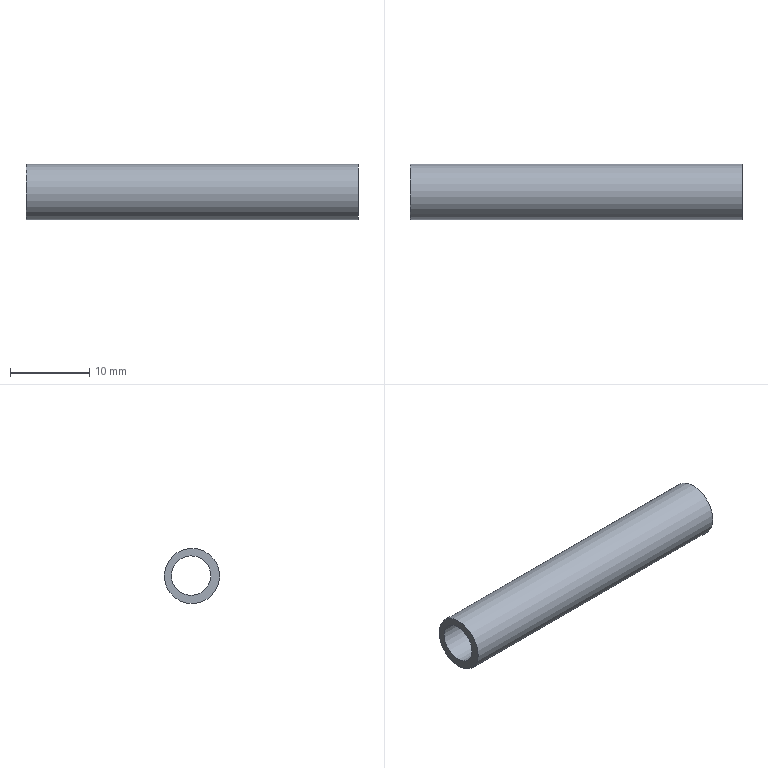Component | NX | 23F__27 | 1 solid | 4 faces | box 42 x 7 x 7 mm | volume 792 mm3 | cylinder 2 | plane 2 | commonest cylinder face diameters 7 x1 5 x1
STEP:
#1=CARTESIAN_POINT('',(0.,0.,0.));
#2=DIRECTION('',(0.,0.,1.));
#3=DIRECTION('',(1.,0.,0.));
#4=AXIS2_PLACEMENT_3D('',#1,#2,#3);
#5=CARTESIAN_POINT('',(87.522,47.062,142.252));
#6=VERTEX_POINT('',#5);
#7=CARTESIAN_POINT('',(87.522,45.581,145.424));
#8=DIRECTION('',(1.,0.,0.));
#9=DIRECTION('',(0.,0.4231,-0.9061));
#10=AXIS2_PLACEMENT_3D('',#7,#8,#9);
#11=CIRCLE('',#10,3.5);
#12=CARTESIAN_POINT('',(87.522,45.581,145.424));
#13=DIRECTION('',(-1.,0.,0.));
#14=DIRECTION('',(0.,-0.4231,0.9061));
#15=AXIS2_PLACEMENT_3D('',#12,#13,#14);
#16=CYLINDRICAL_SURFACE('',#15,3.5);
#17=CARTESIAN_POINT('',(9.425,0.));
#18=DIRECTION('',(-1.,0.));
#19=VECTOR('',#18,1.);
#20=LINE('',#17,#19);
#21=(GEOMETRIC_REPRESENTATION_CONTEXT(2)PARAMETRIC_REPRESENTATION_CONTEXT()REPRESENTATION_CONTEXT('',''));
#22=DEFINITIONAL_REPRESENTATION('',(#20),#21);
#23=PCURVE('',#16,#22);
#24=CARTESIAN_POINT('',(87.522,45.639,145.451));
#25=DIRECTION('',(1.,0.,0.));
#26=DIRECTION('',(0.,0.4231,-0.9061));
#27=AXIS2_PLACEMENT_3D('',#24,#25,#26);
#28=PLANE('',#27);
#29=CARTESIAN_POINT('',(0.,-0.06341));
#30=DIRECTION('',(1.,0.));
#31=AXIS2_PLACEMENT_2D('',#29,#30);
#32=CIRCLE('',#31,3.5);
#33=(GEOMETRIC_REPRESENTATION_CONTEXT(2)PARAMETRIC_REPRESENTATION_CONTEXT()REPRESENTATION_CONTEXT('',''));
#34=DEFINITIONAL_REPRESENTATION('',(#32),#33);
#35=PCURVE('',#28,#34);
#36=SURFACE_CURVE('',#11,(#23,#35),.PCURVE_S1.);
#37=EDGE_CURVE('',#6,#6,#36,.T.);
#38=ORIENTED_EDGE('',*,*,#37,.F.);
#39=CARTESIAN_POINT('',(45.522,47.062,142.252));
#40=VERTEX_POINT('',#39);
#41=CARTESIAN_POINT('',(87.522,47.062,142.252));
#42=CARTESIAN_POINT('',(45.522,47.062,142.252));
#43=B_SPLINE_CURVE_WITH_KNOTS('',1,(#41,#42),.UNSPECIFIED.,.F.,.F.,(2,2),(0.,42.),.PIECEWISE_BEZIER_KNOTS.);
#44=CARTESIAN_POINT('',(9.425,0.));
#45=DIRECTION('',(0.,1.));
#46=VECTOR('',#45,1.);
#47=LINE('',#44,#46);
#48=(GEOMETRIC_REPRESENTATION_CONTEXT(2)PARAMETRIC_REPRESENTATION_CONTEXT()REPRESENTATION_CONTEXT('',''));
#49=DEFINITIONAL_REPRESENTATION('',(#47),#48);
#50=PCURVE('',#16,#49);
#51=CARTESIAN_POINT('',(3.142,0.));
#52=DIRECTION('',(0.,1.));
#53=VECTOR('',#52,1.);
#54=LINE('',#51,#53);
#55=(GEOMETRIC_REPRESENTATION_CONTEXT(2)PARAMETRIC_REPRESENTATION_CONTEXT()REPRESENTATION_CONTEXT('',''));
#56=DEFINITIONAL_REPRESENTATION('',(#54),#55);
#57=PCURVE('',#16,#56);
#58=SEAM_CURVE('',#43,(#50,#57),.PCURVE_S1.);
#59=EDGE_CURVE('',#6,#40,#58,.T.);
#60=ORIENTED_EDGE('',*,*,#59,.T.);
#61=CARTESIAN_POINT('',(45.522,45.581,145.424));
#62=DIRECTION('',(1.,0.,0.));
#63=DIRECTION('',(0.,0.4231,-0.9061));
#64=AXIS2_PLACEMENT_3D('',#61,#62,#63);
#65=CIRCLE('',#64,3.5);
#66=CARTESIAN_POINT('',(9.425,42.));
#67=DIRECTION('',(-1.,0.));
#68=VECTOR('',#67,1.);
#69=LINE('',#66,#68);
#70=(GEOMETRIC_REPRESENTATION_CONTEXT(2)PARAMETRIC_REPRESENTATION_CONTEXT()REPRESENTATION_CONTEXT('',''));
#71=DEFINITIONAL_REPRESENTATION('',(#69),#70);
#72=PCURVE('',#16,#71);
#73=CARTESIAN_POINT('',(45.522,45.639,145.451));
#74=DIRECTION('',(1.,0.,0.));
#75=DIRECTION('',(0.,0.4231,-0.9061));
#76=AXIS2_PLACEMENT_3D('',#73,#74,#75);
#77=PLANE('',#76);
#78=CARTESIAN_POINT('',(0.,-0.06341));
#79=DIRECTION('',(1.,0.));
#80=AXIS2_PLACEMENT_2D('',#78,#79);
#81=CIRCLE('',#80,3.5);
#82=(GEOMETRIC_REPRESENTATION_CONTEXT(2)PARAMETRIC_REPRESENTATION_CONTEXT()REPRESENTATION_CONTEXT('',''));
#83=DEFINITIONAL_REPRESENTATION('',(#81),#82);
#84=PCURVE('',#77,#83);
#85=SURFACE_CURVE('',#65,(#72,#84),.PCURVE_S1.);
#86=EDGE_CURVE('',#40,#40,#85,.T.);
#87=ORIENTED_EDGE('',*,*,#86,.T.);
#88=ORIENTED_EDGE('',*,*,#59,.F.);
#89=EDGE_LOOP('',(#38,#60,#87,#88));
#90=FACE_BOUND('',#89,.T.);
#91=ADVANCED_FACE('',(#90),#16,.T.);
#92=CARTESIAN_POINT('',(87.522,46.754,143.212));
#93=VERTEX_POINT('',#92);
#94=CARTESIAN_POINT('',(87.522,45.696,145.477));
#95=DIRECTION('',(-1.,0.,0.));
#96=DIRECTION('',(0.,0.4231,-0.9061));
#97=AXIS2_PLACEMENT_3D('',#94,#95,#96);
#98=CIRCLE('',#97,2.5);
#99=CARTESIAN_POINT('',(87.522,45.696,145.477));
#100=DIRECTION('',(-1.,0.,0.));
#101=DIRECTION('',(0.,-0.4231,0.9061));
#102=AXIS2_PLACEMENT_3D('',#99,#100,#101);
#103=CYLINDRICAL_SURFACE('',#102,2.5);
#104=CARTESIAN_POINT('',(3.142,0.));
#105=DIRECTION('',(1.,0.));
#106=VECTOR('',#105,1.);
#107=LINE('',#104,#106);
#108=(GEOMETRIC_REPRESENTATION_CONTEXT(2)PARAMETRIC_REPRESENTATION_CONTEXT()REPRESENTATION_CONTEXT('',''));
#109=DEFINITIONAL_REPRESENTATION('',(#107),#108);
#110=PCURVE('',#103,#109);
#111=CARTESIAN_POINT('',(2.5,0.06341));
#112=CARTESIAN_POINT('',(2.5,-4.267));
#113=CARTESIAN_POINT('',(-1.25,-2.102));
#114=CARTESIAN_POINT('',(-5.,0.06341));
#115=CARTESIAN_POINT('',(-1.25,2.228));
#116=CARTESIAN_POINT('',(2.5,4.394));
#117=CARTESIAN_POINT('',(2.5,0.06341));
#118=(BOUNDED_CURVE()B_SPLINE_CURVE(2,(#111,#112,#113,#114,#115,#116,#117),.UNSPECIFIED.,.T.,.F.)B_SPLINE_CURVE_WITH_KNOTS((1,2,2,2,2,1),(-2.094,0.,2.094,4.189,6.283,8.378),.UNSPECIFIED.)CURVE()GEOMETRIC_REPRESENTATION_ITEM()RATIONAL_B_SPLINE_CURVE((1.,0.5,1.,0.5,1.,0.5,1.))REPRESENTATION_ITEM(''));
#119=(GEOMETRIC_REPRESENTATION_CONTEXT(2)PARAMETRIC_REPRESENTATION_CONTEXT()REPRESENTATION_CONTEXT('',''));
#120=DEFINITIONAL_REPRESENTATION('',(#118),#119);
#121=PCURVE('',#28,#120);
#122=SURFACE_CURVE('',#98,(#110,#121),.PCURVE_S1.);
#123=EDGE_CURVE('',#93,#93,#122,.T.);
#124=ORIENTED_EDGE('',*,*,#123,.T.);
#125=CARTESIAN_POINT('',(45.522,46.754,143.212));
#126=VERTEX_POINT('',#125);
#127=CARTESIAN_POINT('',(87.522,46.754,143.212));
#128=CARTESIAN_POINT('',(45.522,46.754,143.212));
#129=B_SPLINE_CURVE_WITH_KNOTS('',1,(#127,#128),.UNSPECIFIED.,.F.,.F.,(2,2),(0.,42.),.PIECEWISE_BEZIER_KNOTS.);
#130=CARTESIAN_POINT('',(9.425,0.));
#131=DIRECTION('',(0.,1.));
#132=VECTOR('',#131,1.);
#133=LINE('',#130,#132);
#134=(GEOMETRIC_REPRESENTATION_CONTEXT(2)PARAMETRIC_REPRESENTATION_CONTEXT()REPRESENTATION_CONTEXT('',''));
#135=DEFINITIONAL_REPRESENTATION('',(#133),#134);
#136=PCURVE('',#103,#135);
#137=CARTESIAN_POINT('',(3.142,0.));
#138=DIRECTION('',(0.,1.));
#139=VECTOR('',#138,1.);
#140=LINE('',#137,#139);
#141=(GEOMETRIC_REPRESENTATION_CONTEXT(2)PARAMETRIC_REPRESENTATION_CONTEXT()REPRESENTATION_CONTEXT('',''));
#142=DEFINITIONAL_REPRESENTATION('',(#140),#141);
#143=PCURVE('',#103,#142);
#144=SEAM_CURVE('',#129,(#136,#143),.PCURVE_S1.);
#145=EDGE_CURVE('',#93,#126,#144,.T.);
#146=ORIENTED_EDGE('',*,*,#145,.T.);
#147=CARTESIAN_POINT('',(45.522,45.696,145.477));
#148=DIRECTION('',(-1.,0.,0.));
#149=DIRECTION('',(0.,0.4231,-0.9061));
#150=AXIS2_PLACEMENT_3D('',#147,#148,#149);
#151=CIRCLE('',#150,2.5);
#152=CARTESIAN_POINT('',(3.142,42.));
#153=DIRECTION('',(1.,0.));
#154=VECTOR('',#153,1.);
#155=LINE('',#152,#154);
#156=(GEOMETRIC_REPRESENTATION_CONTEXT(2)PARAMETRIC_REPRESENTATION_CONTEXT()REPRESENTATION_CONTEXT('',''));
#157=DEFINITIONAL_REPRESENTATION('',(#155),#156);
#158=PCURVE('',#103,#157);
#159=CARTESIAN_POINT('',(2.5,0.06341));
#160=CARTESIAN_POINT('',(2.5,-4.267));
#161=CARTESIAN_POINT('',(-1.25,-2.102));
#162=CARTESIAN_POINT('',(-5.,0.06341));
#163=CARTESIAN_POINT('',(-1.25,2.228));
#164=CARTESIAN_POINT('',(2.5,4.394));
#165=CARTESIAN_POINT('',(2.5,0.06341));
#166=(BOUNDED_CURVE()B_SPLINE_CURVE(2,(#159,#160,#161,#162,#163,#164,#165),.UNSPECIFIED.,.T.,.F.)B_SPLINE_CURVE_WITH_KNOTS((1,2,2,2,2,1),(-2.094,0.,2.094,4.189,6.283,8.378),.UNSPECIFIED.)CURVE()GEOMETRIC_REPRESENTATION_ITEM()RATIONAL_B_SPLINE_CURVE((1.,0.5,1.,0.5,1.,0.5,1.))REPRESENTATION_ITEM(''));
#167=(GEOMETRIC_REPRESENTATION_CONTEXT(2)PARAMETRIC_REPRESENTATION_CONTEXT()REPRESENTATION_CONTEXT('',''));
#168=DEFINITIONAL_REPRESENTATION('',(#166),#167);
#169=PCURVE('',#77,#168);
#170=SURFACE_CURVE('',#151,(#158,#169),.PCURVE_S1.);
#171=EDGE_CURVE('',#126,#126,#170,.T.);
#172=ORIENTED_EDGE('',*,*,#171,.F.);
#173=ORIENTED_EDGE('',*,*,#145,.F.);
#174=EDGE_LOOP('',(#124,#146,#172,#173));
#175=FACE_BOUND('',#174,.F.);
#176=ADVANCED_FACE('',(#175),#103,.F.);
#177=ORIENTED_EDGE('',*,*,#37,.T.);
#178=EDGE_LOOP('',(#177));
#179=FACE_BOUND('',#178,.T.);
#180=ORIENTED_EDGE('',*,*,#123,.T.);
#181=EDGE_LOOP('',(#180));
#182=FACE_BOUND('',#181,.T.);
#183=ADVANCED_FACE('',(#179,#182),#28,.T.);
#184=ORIENTED_EDGE('',*,*,#86,.F.);
#185=EDGE_LOOP('',(#184));
#186=FACE_BOUND('',#185,.T.);
#187=ORIENTED_EDGE('',*,*,#171,.F.);
#188=EDGE_LOOP('',(#187));
#189=FACE_BOUND('',#188,.T.);
#190=ADVANCED_FACE('',(#186,#189),#77,.F.);
#191=CLOSED_SHELL('',(#91,#176,#183,#190));
#192=MANIFOLD_SOLID_BREP('',#191);
#193=(LENGTH_UNIT()NAMED_UNIT(*)SI_UNIT(.MILLI.,.METRE.));
#194=UNCERTAINTY_MEASURE_WITH_UNIT(LENGTH_MEASURE(0.00001),#193,'','');
#195=(NAMED_UNIT(*)PLANE_ANGLE_UNIT()SI_UNIT($,.RADIAN.));
#196=(NAMED_UNIT(*)SI_UNIT($,.STERADIAN.)SOLID_ANGLE_UNIT());
#197=(GEOMETRIC_REPRESENTATION_CONTEXT(3)GLOBAL_UNCERTAINTY_ASSIGNED_CONTEXT((#194))GLOBAL_UNIT_ASSIGNED_CONTEXT((#193,#195,#196))REPRESENTATION_CONTEXT('',''));
#198=ADVANCED_BREP_SHAPE_REPRESENTATION('',(#4,#192),#197);